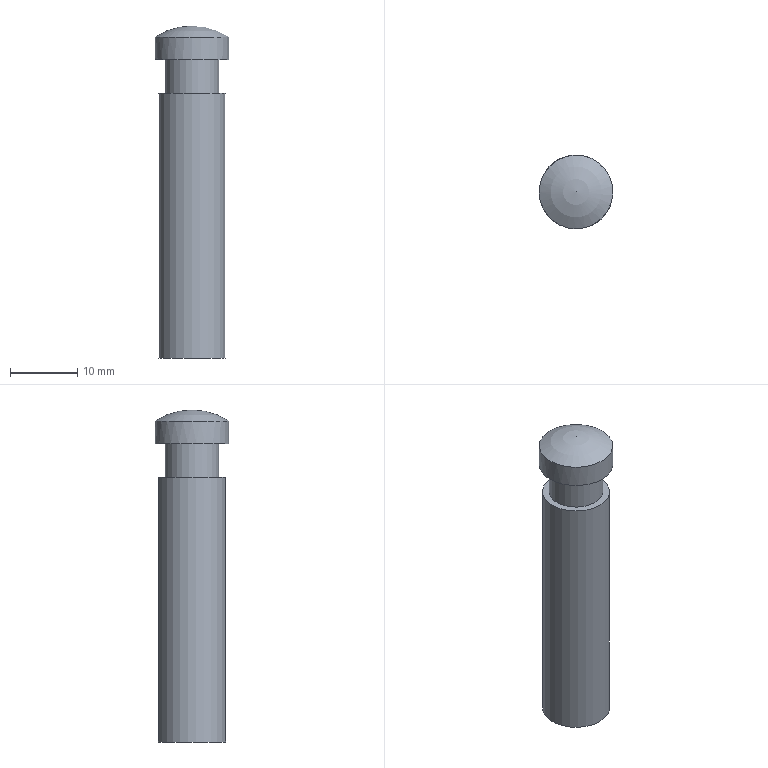Component | NX | B_STUD_2 | 1 solid | 7 faces | box 11 x 11 x 49.5 mm | volume 3753 mm3 | plane 3 | cylinder 3 | sphere 1 | commonest cylinder face diameters 11 x1 8 x1 10 x1
STEP:
#1=CARTESIAN_POINT('',(0.,0.,0.));
#2=DIRECTION('',(0.,0.,1.));
#3=DIRECTION('',(1.,0.,0.));
#4=AXIS2_PLACEMENT_3D('',#1,#2,#3);
#5=CARTESIAN_POINT('',(457.101,-5.,-8.));
#6=VERTEX_POINT('',#5);
#7=CARTESIAN_POINT('',(457.101,0.,-8.));
#8=DIRECTION('',(0.,0.,1.));
#9=DIRECTION('',(0.,-1.,0.));
#10=AXIS2_PLACEMENT_3D('',#7,#8,#9);
#11=CIRCLE('',#10,5.);
#12=CARTESIAN_POINT('',(457.101,0.,-8.));
#13=DIRECTION('',(0.,0.,1.));
#14=DIRECTION('',(0.,-1.,0.));
#15=AXIS2_PLACEMENT_3D('',#12,#13,#14);
#16=PLANE('',#15);
#17=CARTESIAN_POINT('',(0.,0.));
#18=DIRECTION('',(1.,0.));
#19=AXIS2_PLACEMENT_2D('',#17,#18);
#20=CIRCLE('',#19,5.);
#21=(GEOMETRIC_REPRESENTATION_CONTEXT(2)PARAMETRIC_REPRESENTATION_CONTEXT()REPRESENTATION_CONTEXT('',''));
#22=DEFINITIONAL_REPRESENTATION('',(#20),#21);
#23=PCURVE('',#16,#22);
#24=CARTESIAN_POINT('',(457.101,0.,-8.));
#25=DIRECTION('',(0.,0.,1.));
#26=DIRECTION('',(0.,-1.,0.));
#27=AXIS2_PLACEMENT_3D('',#24,#25,#26);
#28=CYLINDRICAL_SURFACE('',#27,5.);
#29=CARTESIAN_POINT('',(0.,0.));
#30=DIRECTION('',(1.,0.));
#31=VECTOR('',#30,1.);
#32=LINE('',#29,#31);
#33=(GEOMETRIC_REPRESENTATION_CONTEXT(2)PARAMETRIC_REPRESENTATION_CONTEXT()REPRESENTATION_CONTEXT('',''));
#34=DEFINITIONAL_REPRESENTATION('',(#32),#33);
#35=PCURVE('',#28,#34);
#36=SURFACE_CURVE('',#11,(#23,#35),.PCURVE_S1.);
#37=EDGE_CURVE('',#6,#6,#36,.T.);
#38=ORIENTED_EDGE('',*,*,#37,.F.);
#39=EDGE_LOOP('',(#38));
#40=FACE_BOUND('',#39,.T.);
#41=ADVANCED_FACE('',(#40),#16,.F.);
#42=CARTESIAN_POINT('',(457.101,-5.5,39.852));
#43=VERTEX_POINT('',#42);
#44=CARTESIAN_POINT('',(451.601,0.,39.852));
#45=VERTEX_POINT('',#44);
#46=CARTESIAN_POINT('',(457.101,0.,39.852));
#47=DIRECTION('',(0.,0.,1.));
#48=DIRECTION('',(0.,-1.,0.));
#49=AXIS2_PLACEMENT_3D('',#46,#47,#48);
#50=CIRCLE('',#49,5.5);
#51=CARTESIAN_POINT('',(457.101,0.,31.5));
#52=DIRECTION('',(0.,0.,1.));
#53=DIRECTION('',(-1.,0.,0.));
#54=AXIS2_PLACEMENT_3D('',#51,#52,#53);
#55=SPHERICAL_SURFACE('',#54,10.);
#56=CARTESIAN_POINT('',(1.571,0.9884));
#57=CARTESIAN_POINT('',(1.666,0.9884));
#58=CARTESIAN_POINT('',(1.856,0.9884));
#59=CARTESIAN_POINT('',(2.142,0.9884));
#60=CARTESIAN_POINT('',(2.428,0.9884));
#61=CARTESIAN_POINT('',(2.713,0.9884));
#62=CARTESIAN_POINT('',(2.999,0.9884));
#63=CARTESIAN_POINT('',(3.284,0.9884));
#64=CARTESIAN_POINT('',(3.57,0.9884));
#65=CARTESIAN_POINT('',(3.856,0.9884));
#66=CARTESIAN_POINT('',(4.141,0.9884));
#67=CARTESIAN_POINT('',(4.427,0.9884));
#68=CARTESIAN_POINT('',(4.712,0.9884));
#69=CARTESIAN_POINT('',(4.998,0.9884));
#70=CARTESIAN_POINT('',(5.284,0.9884));
#71=CARTESIAN_POINT('',(5.569,0.9884));
#72=CARTESIAN_POINT('',(5.855,0.9884));
#73=CARTESIAN_POINT('',(6.14,0.9884));
#74=CARTESIAN_POINT('',(6.426,0.9884));
#75=CARTESIAN_POINT('',(6.712,0.9884));
#76=CARTESIAN_POINT('',(6.997,0.9884));
#77=CARTESIAN_POINT('',(7.283,0.9884));
#78=CARTESIAN_POINT('',(7.568,0.9884));
#79=CARTESIAN_POINT('',(7.759,0.9884));
#80=CARTESIAN_POINT('',(7.854,0.9884));
#81=B_SPLINE_CURVE_WITH_KNOTS('',3,(#56,#57,#58,#59,#60,#61,#62,#63,#64,#65,#66,#67,#68,#69,#70,#71,#72,#73,#74,#75,#76,#77,#78,#79,#80),.UNSPECIFIED.,.F.,.F.,(4,1,1,1,1,1,1,1,1,1,1,1,1,1,1,1,1,1,1,1,1,1,4),(0.,0.2856,0.5712,0.8568,1.142,1.428,1.714,1.999,2.285,2.57,2.856,3.142,3.427,3.713,3.998,4.284,4.57,4.855,5.141,5.426,5.712,5.998,6.283),.QUASI_UNIFORM_KNOTS.);
#82=(GEOMETRIC_REPRESENTATION_CONTEXT(2)PARAMETRIC_REPRESENTATION_CONTEXT()REPRESENTATION_CONTEXT('',''));
#83=DEFINITIONAL_REPRESENTATION('',(#81),#82);
#84=PCURVE('',#55,#83);
#85=CARTESIAN_POINT('',(457.101,0.,-8.));
#86=DIRECTION('',(0.,0.,1.));
#87=DIRECTION('',(0.,-1.,0.));
#88=AXIS2_PLACEMENT_3D('',#85,#86,#87);
#89=CYLINDRICAL_SURFACE('',#88,5.5);
#90=CARTESIAN_POINT('',(0.,47.852));
#91=DIRECTION('',(1.,0.));
#92=VECTOR('',#91,1.);
#93=LINE('',#90,#92);
#94=(GEOMETRIC_REPRESENTATION_CONTEXT(2)PARAMETRIC_REPRESENTATION_CONTEXT()REPRESENTATION_CONTEXT('',''));
#95=DEFINITIONAL_REPRESENTATION('',(#93),#94);
#96=PCURVE('',#89,#95);
#97=SURFACE_CURVE('',#50,(#84,#96),.PCURVE_S1.);
#98=EDGE_CURVE('',#43,#45,#97,.T.);
#99=ORIENTED_EDGE('',*,*,#98,.T.);
#100=CARTESIAN_POINT('',(457.101,0.,41.5));
#101=VERTEX_POINT('',#100);
#102=CARTESIAN_POINT('',(451.601,0.,39.852));
#103=CARTESIAN_POINT('',(452.574,0.,40.492));
#104=CARTESIAN_POINT('',(453.64,0.,40.991));
#105=CARTESIAN_POINT('',(454.772,0.,41.33));
#106=CARTESIAN_POINT('',(455.936,0.,41.5));
#107=CARTESIAN_POINT('',(457.101,0.,41.5));
#108=B_SPLINE_CURVE_WITH_KNOTS('',5,(#102,#103,#104,#105,#106,#107),.UNSPECIFIED.,.F.,.F.,(6,6),(0.9884,1.571),.PIECEWISE_BEZIER_KNOTS.);
#109=CARTESIAN_POINT('',(6.283,0.));
#110=DIRECTION('',(0.,1.));
#111=VECTOR('',#110,1.);
#112=LINE('',#109,#111);
#113=(GEOMETRIC_REPRESENTATION_CONTEXT(2)PARAMETRIC_REPRESENTATION_CONTEXT()REPRESENTATION_CONTEXT('',''));
#114=DEFINITIONAL_REPRESENTATION('',(#112),#113);
#115=PCURVE('',#55,#114);
#116=CARTESIAN_POINT('',(0.,0.));
#117=DIRECTION('',(0.,1.));
#118=VECTOR('',#117,1.);
#119=LINE('',#116,#118);
#120=(GEOMETRIC_REPRESENTATION_CONTEXT(2)PARAMETRIC_REPRESENTATION_CONTEXT()REPRESENTATION_CONTEXT('',''));
#121=DEFINITIONAL_REPRESENTATION('',(#119),#120);
#122=PCURVE('',#55,#121);
#123=SEAM_CURVE('',#108,(#115,#122),.PCURVE_S1.);
#124=EDGE_CURVE('',#45,#101,#123,.T.);
#125=ORIENTED_EDGE('',*,*,#124,.T.);
#126=ORIENTED_EDGE('',*,*,#124,.F.);
#127=CARTESIAN_POINT('',(457.101,0.,39.852));
#128=DIRECTION('',(0.,0.,1.));
#129=DIRECTION('',(0.,-1.,0.));
#130=AXIS2_PLACEMENT_3D('',#127,#128,#129);
#131=CIRCLE('',#130,5.5);
#132=CARTESIAN_POINT('',(-4.712,0.9884));
#133=CARTESIAN_POINT('',(-4.617,0.9884));
#134=CARTESIAN_POINT('',(-4.427,0.9884));
#135=CARTESIAN_POINT('',(-4.141,0.9884));
#136=CARTESIAN_POINT('',(-3.856,0.9884));
#137=CARTESIAN_POINT('',(-3.57,0.9884));
#138=CARTESIAN_POINT('',(-3.284,0.9884));
#139=CARTESIAN_POINT('',(-2.999,0.9884));
#140=CARTESIAN_POINT('',(-2.713,0.9884));
#141=CARTESIAN_POINT('',(-2.428,0.9884));
#142=CARTESIAN_POINT('',(-2.142,0.9884));
#143=CARTESIAN_POINT('',(-1.856,0.9884));
#144=CARTESIAN_POINT('',(-1.571,0.9884));
#145=CARTESIAN_POINT('',(-1.285,0.9884));
#146=CARTESIAN_POINT('',(-0.9996,0.9884));
#147=CARTESIAN_POINT('',(-0.714,0.9884));
#148=CARTESIAN_POINT('',(-0.4284,0.9884));
#149=CARTESIAN_POINT('',(-0.1428,0.9884));
#150=CARTESIAN_POINT('',(0.1428,0.9884));
#151=CARTESIAN_POINT('',(0.4284,0.9884));
#152=CARTESIAN_POINT('',(0.714,0.9884));
#153=CARTESIAN_POINT('',(0.9996,0.9884));
#154=CARTESIAN_POINT('',(1.285,0.9884));
#155=CARTESIAN_POINT('',(1.476,0.9884));
#156=CARTESIAN_POINT('',(1.571,0.9884));
#157=B_SPLINE_CURVE_WITH_KNOTS('',3,(#132,#133,#134,#135,#136,#137,#138,#139,#140,#141,#142,#143,#144,#145,#146,#147,#148,#149,#150,#151,#152,#153,#154,#155,#156),.UNSPECIFIED.,.F.,.F.,(4,1,1,1,1,1,1,1,1,1,1,1,1,1,1,1,1,1,1,1,1,1,4),(0.,0.2856,0.5712,0.8568,1.142,1.428,1.714,1.999,2.285,2.57,2.856,3.142,3.427,3.713,3.998,4.284,4.57,4.855,5.141,5.426,5.712,5.998,6.283),.QUASI_UNIFORM_KNOTS.);
#158=(GEOMETRIC_REPRESENTATION_CONTEXT(2)PARAMETRIC_REPRESENTATION_CONTEXT()REPRESENTATION_CONTEXT('',''));
#159=DEFINITIONAL_REPRESENTATION('',(#157),#158);
#160=PCURVE('',#55,#159);
#161=CARTESIAN_POINT('',(0.,47.852));
#162=DIRECTION('',(1.,0.));
#163=VECTOR('',#162,1.);
#164=LINE('',#161,#163);
#165=(GEOMETRIC_REPRESENTATION_CONTEXT(2)PARAMETRIC_REPRESENTATION_CONTEXT()REPRESENTATION_CONTEXT('',''));
#166=DEFINITIONAL_REPRESENTATION('',(#164),#165);
#167=PCURVE('',#89,#166);
#168=SURFACE_CURVE('',#131,(#160,#167),.PCURVE_S1.);
#169=EDGE_CURVE('',#45,#43,#168,.T.);
#170=ORIENTED_EDGE('',*,*,#169,.T.);
#171=EDGE_LOOP('',(#99,#125,#126,#170));
#172=FACE_BOUND('',#171,.T.);
#173=ADVANCED_FACE('',(#172),#55,.T.);
#174=ORIENTED_EDGE('',*,*,#98,.F.);
#175=CARTESIAN_POINT('',(457.101,-5.5,36.5));
#176=VERTEX_POINT('',#175);
#177=CARTESIAN_POINT('',(457.101,-5.5,36.5));
#178=CARTESIAN_POINT('',(457.101,-5.5,39.852));
#179=B_SPLINE_CURVE_WITH_KNOTS('',1,(#177,#178),.UNSPECIFIED.,.F.,.F.,(2,2),(44.5,47.852),.PIECEWISE_BEZIER_KNOTS.);
#180=CARTESIAN_POINT('',(0.,0.));
#181=DIRECTION('',(0.,1.));
#182=VECTOR('',#181,1.);
#183=LINE('',#180,#182);
#184=(GEOMETRIC_REPRESENTATION_CONTEXT(2)PARAMETRIC_REPRESENTATION_CONTEXT()REPRESENTATION_CONTEXT('',''));
#185=DEFINITIONAL_REPRESENTATION('',(#183),#184);
#186=PCURVE('',#89,#185);
#187=CARTESIAN_POINT('',(6.283,0.));
#188=DIRECTION('',(0.,1.));
#189=VECTOR('',#188,1.);
#190=LINE('',#187,#189);
#191=(GEOMETRIC_REPRESENTATION_CONTEXT(2)PARAMETRIC_REPRESENTATION_CONTEXT()REPRESENTATION_CONTEXT('',''));
#192=DEFINITIONAL_REPRESENTATION('',(#190),#191);
#193=PCURVE('',#89,#192);
#194=SEAM_CURVE('',#179,(#186,#193),.PCURVE_S1.);
#195=EDGE_CURVE('',#176,#43,#194,.T.);
#196=ORIENTED_EDGE('',*,*,#195,.F.);
#197=CARTESIAN_POINT('',(457.101,0.,36.5));
#198=DIRECTION('',(0.,0.,1.));
#199=DIRECTION('',(0.,-1.,0.));
#200=AXIS2_PLACEMENT_3D('',#197,#198,#199);
#201=CIRCLE('',#200,5.5);
#202=CARTESIAN_POINT('',(0.,44.5));
#203=DIRECTION('',(1.,0.));
#204=VECTOR('',#203,1.);
#205=LINE('',#202,#204);
#206=(GEOMETRIC_REPRESENTATION_CONTEXT(2)PARAMETRIC_REPRESENTATION_CONTEXT()REPRESENTATION_CONTEXT('',''));
#207=DEFINITIONAL_REPRESENTATION('',(#205),#206);
#208=PCURVE('',#89,#207);
#209=CARTESIAN_POINT('',(453.101,0.,36.5));
#210=DIRECTION('',(0.,0.,1.));
#211=DIRECTION('',(0.,-1.,0.));
#212=AXIS2_PLACEMENT_3D('',#209,#210,#211);
#213=PLANE('',#212);
#214=CARTESIAN_POINT('',(0.,4.));
#215=DIRECTION('',(1.,0.));
#216=AXIS2_PLACEMENT_2D('',#214,#215);
#217=CIRCLE('',#216,5.5);
#218=(GEOMETRIC_REPRESENTATION_CONTEXT(2)PARAMETRIC_REPRESENTATION_CONTEXT()REPRESENTATION_CONTEXT('',''));
#219=DEFINITIONAL_REPRESENTATION('',(#217),#218);
#220=PCURVE('',#213,#219);
#221=SURFACE_CURVE('',#201,(#208,#220),.PCURVE_S1.);
#222=EDGE_CURVE('',#176,#176,#221,.T.);
#223=ORIENTED_EDGE('',*,*,#222,.T.);
#224=ORIENTED_EDGE('',*,*,#195,.T.);
#225=ORIENTED_EDGE('',*,*,#169,.F.);
#226=EDGE_LOOP('',(#174,#196,#223,#224,#225));
#227=FACE_BOUND('',#226,.T.);
#228=ADVANCED_FACE('',(#227),#89,.T.);
#229=ORIENTED_EDGE('',*,*,#222,.F.);
#230=EDGE_LOOP('',(#229));
#231=FACE_BOUND('',#230,.T.);
#232=CARTESIAN_POINT('',(457.101,-4.,36.5));
#233=VERTEX_POINT('',#232);
#234=CARTESIAN_POINT('',(457.101,0.,36.5));
#235=DIRECTION('',(0.,0.,1.));
#236=DIRECTION('',(0.,-1.,0.));
#237=AXIS2_PLACEMENT_3D('',#234,#235,#236);
#238=CIRCLE('',#237,4.);
#239=CARTESIAN_POINT('',(0.,4.));
#240=DIRECTION('',(1.,0.));
#241=AXIS2_PLACEMENT_2D('',#239,#240);
#242=CIRCLE('',#241,4.);
#243=(GEOMETRIC_REPRESENTATION_CONTEXT(2)PARAMETRIC_REPRESENTATION_CONTEXT()REPRESENTATION_CONTEXT('',''));
#244=DEFINITIONAL_REPRESENTATION('',(#242),#243);
#245=PCURVE('',#213,#244);
#246=CARTESIAN_POINT('',(457.101,0.,-8.));
#247=DIRECTION('',(0.,0.,1.));
#248=DIRECTION('',(0.,-1.,0.));
#249=AXIS2_PLACEMENT_3D('',#246,#247,#248);
#250=CYLINDRICAL_SURFACE('',#249,4.);
#251=CARTESIAN_POINT('',(0.,44.5));
#252=DIRECTION('',(1.,0.));
#253=VECTOR('',#252,1.);
#254=LINE('',#251,#253);
#255=(GEOMETRIC_REPRESENTATION_CONTEXT(2)PARAMETRIC_REPRESENTATION_CONTEXT()REPRESENTATION_CONTEXT('',''));
#256=DEFINITIONAL_REPRESENTATION('',(#254),#255);
#257=PCURVE('',#250,#256);
#258=SURFACE_CURVE('',#238,(#245,#257),.PCURVE_S1.);
#259=EDGE_CURVE('',#233,#233,#258,.T.);
#260=ORIENTED_EDGE('',*,*,#259,.T.);
#261=EDGE_LOOP('',(#260));
#262=FACE_BOUND('',#261,.T.);
#263=ADVANCED_FACE('',(#231,#262),#213,.F.);
#264=ORIENTED_EDGE('',*,*,#259,.F.);
#265=CARTESIAN_POINT('',(457.101,-4.,31.5));
#266=VERTEX_POINT('',#265);
#267=CARTESIAN_POINT('',(457.101,-4.,31.5));
#268=CARTESIAN_POINT('',(457.101,-4.,36.5));
#269=B_SPLINE_CURVE_WITH_KNOTS('',1,(#267,#268),.UNSPECIFIED.,.F.,.F.,(2,2),(39.5,44.5),.PIECEWISE_BEZIER_KNOTS.);
#270=CARTESIAN_POINT('',(0.,0.));
#271=DIRECTION('',(0.,1.));
#272=VECTOR('',#271,1.);
#273=LINE('',#270,#272);
#274=(GEOMETRIC_REPRESENTATION_CONTEXT(2)PARAMETRIC_REPRESENTATION_CONTEXT()REPRESENTATION_CONTEXT('',''));
#275=DEFINITIONAL_REPRESENTATION('',(#273),#274);
#276=PCURVE('',#250,#275);
#277=CARTESIAN_POINT('',(6.283,0.));
#278=DIRECTION('',(0.,1.));
#279=VECTOR('',#278,1.);
#280=LINE('',#277,#279);
#281=(GEOMETRIC_REPRESENTATION_CONTEXT(2)PARAMETRIC_REPRESENTATION_CONTEXT()REPRESENTATION_CONTEXT('',''));
#282=DEFINITIONAL_REPRESENTATION('',(#280),#281);
#283=PCURVE('',#250,#282);
#284=SEAM_CURVE('',#269,(#276,#283),.PCURVE_S1.);
#285=EDGE_CURVE('',#266,#233,#284,.T.);
#286=ORIENTED_EDGE('',*,*,#285,.F.);
#287=CARTESIAN_POINT('',(457.101,0.,31.5));
#288=DIRECTION('',(0.,0.,1.));
#289=DIRECTION('',(0.,-1.,0.));
#290=AXIS2_PLACEMENT_3D('',#287,#288,#289);
#291=CIRCLE('',#290,4.);
#292=CARTESIAN_POINT('',(0.,39.5));
#293=DIRECTION('',(1.,0.));
#294=VECTOR('',#293,1.);
#295=LINE('',#292,#294);
#296=(GEOMETRIC_REPRESENTATION_CONTEXT(2)PARAMETRIC_REPRESENTATION_CONTEXT()REPRESENTATION_CONTEXT('',''));
#297=DEFINITIONAL_REPRESENTATION('',(#295),#296);
#298=PCURVE('',#250,#297);
#299=CARTESIAN_POINT('',(452.101,0.,31.5));
#300=DIRECTION('',(0.,0.,-1.));
#301=DIRECTION('',(0.,1.,0.));
#302=AXIS2_PLACEMENT_3D('',#299,#300,#301);
#303=PLANE('',#302);
#304=CARTESIAN_POINT('',(-4.,5.));
#305=CARTESIAN_POINT('',(-4.,11.928));
#306=CARTESIAN_POINT('',(2.,8.464));
#307=CARTESIAN_POINT('',(8.,5.));
#308=CARTESIAN_POINT('',(2.,1.536));
#309=CARTESIAN_POINT('',(-4.,-1.928));
#310=CARTESIAN_POINT('',(-4.,5.));
#311=(BOUNDED_CURVE()B_SPLINE_CURVE(2,(#304,#305,#306,#307,#308,#309,#310),.UNSPECIFIED.,.T.,.F.)B_SPLINE_CURVE_WITH_KNOTS((1,2,2,2,2,1),(-2.094,0.,2.094,4.189,6.283,8.378),.UNSPECIFIED.)CURVE()GEOMETRIC_REPRESENTATION_ITEM()RATIONAL_B_SPLINE_CURVE((1.,0.5,1.,0.5,1.,0.5,1.))REPRESENTATION_ITEM(''));
#312=(GEOMETRIC_REPRESENTATION_CONTEXT(2)PARAMETRIC_REPRESENTATION_CONTEXT()REPRESENTATION_CONTEXT('',''));
#313=DEFINITIONAL_REPRESENTATION('',(#311),#312);
#314=PCURVE('',#303,#313);
#315=SURFACE_CURVE('',#291,(#298,#314),.PCURVE_S1.);
#316=EDGE_CURVE('',#266,#266,#315,.T.);
#317=ORIENTED_EDGE('',*,*,#316,.T.);
#318=ORIENTED_EDGE('',*,*,#285,.T.);
#319=EDGE_LOOP('',(#264,#286,#317,#318));
#320=FACE_BOUND('',#319,.T.);
#321=ADVANCED_FACE('',(#320),#250,.T.);
#322=ORIENTED_EDGE('',*,*,#316,.F.);
#323=EDGE_LOOP('',(#322));
#324=FACE_BOUND('',#323,.T.);
#325=CARTESIAN_POINT('',(457.101,-5.,31.5));
#326=VERTEX_POINT('',#325);
#327=CARTESIAN_POINT('',(457.101,0.,31.5));
#328=DIRECTION('',(0.,0.,1.));
#329=DIRECTION('',(0.,-1.,0.));
#330=AXIS2_PLACEMENT_3D('',#327,#328,#329);
#331=CIRCLE('',#330,5.);
#332=CARTESIAN_POINT('',(-5.,5.));
#333=CARTESIAN_POINT('',(-5.,13.66));
#334=CARTESIAN_POINT('',(2.5,9.33));
#335=CARTESIAN_POINT('',(10.,5.));
#336=CARTESIAN_POINT('',(2.5,0.6699));
#337=CARTESIAN_POINT('',(-5.,-3.66));
#338=CARTESIAN_POINT('',(-5.,5.));
#339=(BOUNDED_CURVE()B_SPLINE_CURVE(2,(#332,#333,#334,#335,#336,#337,#338),.UNSPECIFIED.,.T.,.F.)B_SPLINE_CURVE_WITH_KNOTS((1,2,2,2,2,1),(-2.094,0.,2.094,4.189,6.283,8.378),.UNSPECIFIED.)CURVE()GEOMETRIC_REPRESENTATION_ITEM()RATIONAL_B_SPLINE_CURVE((1.,0.5,1.,0.5,1.,0.5,1.))REPRESENTATION_ITEM(''));
#340=(GEOMETRIC_REPRESENTATION_CONTEXT(2)PARAMETRIC_REPRESENTATION_CONTEXT()REPRESENTATION_CONTEXT('',''));
#341=DEFINITIONAL_REPRESENTATION('',(#339),#340);
#342=PCURVE('',#303,#341);
#343=CARTESIAN_POINT('',(0.,39.5));
#344=DIRECTION('',(1.,0.));
#345=VECTOR('',#344,1.);
#346=LINE('',#343,#345);
#347=(GEOMETRIC_REPRESENTATION_CONTEXT(2)PARAMETRIC_REPRESENTATION_CONTEXT()REPRESENTATION_CONTEXT('',''));
#348=DEFINITIONAL_REPRESENTATION('',(#346),#347);
#349=PCURVE('',#28,#348);
#350=SURFACE_CURVE('',#331,(#342,#349),.PCURVE_S1.);
#351=EDGE_CURVE('',#326,#326,#350,.T.);
#352=ORIENTED_EDGE('',*,*,#351,.T.);
#353=EDGE_LOOP('',(#352));
#354=FACE_BOUND('',#353,.T.);
#355=ADVANCED_FACE('',(#324,#354),#303,.F.);
#356=ORIENTED_EDGE('',*,*,#351,.F.);
#357=CARTESIAN_POINT('',(457.101,-5.,-8.));
#358=CARTESIAN_POINT('',(457.101,-5.,31.5));
#359=B_SPLINE_CURVE_WITH_KNOTS('',1,(#357,#358),.UNSPECIFIED.,.F.,.F.,(2,2),(0.,39.5),.PIECEWISE_BEZIER_KNOTS.);
#360=CARTESIAN_POINT('',(0.,0.));
#361=DIRECTION('',(0.,1.));
#362=VECTOR('',#361,1.);
#363=LINE('',#360,#362);
#364=(GEOMETRIC_REPRESENTATION_CONTEXT(2)PARAMETRIC_REPRESENTATION_CONTEXT()REPRESENTATION_CONTEXT('',''));
#365=DEFINITIONAL_REPRESENTATION('',(#363),#364);
#366=PCURVE('',#28,#365);
#367=CARTESIAN_POINT('',(6.283,0.));
#368=DIRECTION('',(0.,1.));
#369=VECTOR('',#368,1.);
#370=LINE('',#367,#369);
#371=(GEOMETRIC_REPRESENTATION_CONTEXT(2)PARAMETRIC_REPRESENTATION_CONTEXT()REPRESENTATION_CONTEXT('',''));
#372=DEFINITIONAL_REPRESENTATION('',(#370),#371);
#373=PCURVE('',#28,#372);
#374=SEAM_CURVE('',#359,(#366,#373),.PCURVE_S1.);
#375=EDGE_CURVE('',#6,#326,#374,.T.);
#376=ORIENTED_EDGE('',*,*,#375,.F.);
#377=ORIENTED_EDGE('',*,*,#37,.T.);
#378=ORIENTED_EDGE('',*,*,#375,.T.);
#379=EDGE_LOOP('',(#356,#376,#377,#378));
#380=FACE_BOUND('',#379,.T.);
#381=ADVANCED_FACE('',(#380),#28,.T.);
#382=CLOSED_SHELL('',(#41,#173,#228,#263,#321,#355,#381));
#383=MANIFOLD_SOLID_BREP('',#382);
#384=(LENGTH_UNIT()NAMED_UNIT(*)SI_UNIT(.MILLI.,.METRE.));
#385=UNCERTAINTY_MEASURE_WITH_UNIT(LENGTH_MEASURE(0.00001),#384,'','');
#386=(NAMED_UNIT(*)PLANE_ANGLE_UNIT()SI_UNIT($,.RADIAN.));
#387=(NAMED_UNIT(*)SI_UNIT($,.STERADIAN.)SOLID_ANGLE_UNIT());
#388=(GEOMETRIC_REPRESENTATION_CONTEXT(3)GLOBAL_UNCERTAINTY_ASSIGNED_CONTEXT((#385))GLOBAL_UNIT_ASSIGNED_CONTEXT((#384,#386,#387))REPRESENTATION_CONTEXT('',''));
#389=ADVANCED_BREP_SHAPE_REPRESENTATION('',(#4,#383),#388);